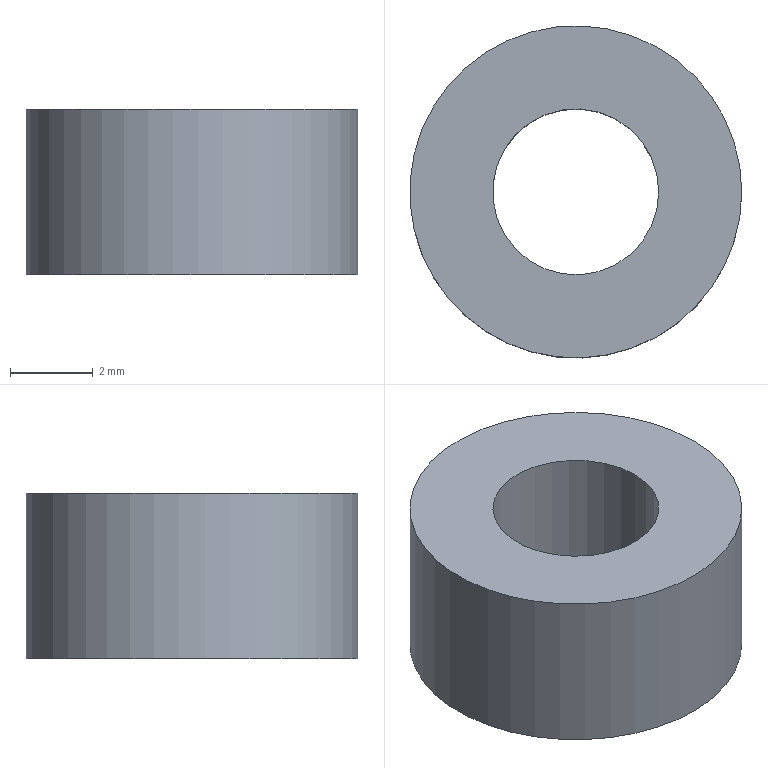Component | NX | LARGE_WASHER | 1 solid | 4 faces | box 8 x 8 x 4 mm | volume 151 mm3 | cylinder 2 | plane 2 | commonest cylinder face diameters 8 x1 4 x1
STEP:
#1=CARTESIAN_POINT('',(0.,0.,0.));
#2=DIRECTION('',(0.,0.,1.));
#3=DIRECTION('',(1.,0.,0.));
#4=AXIS2_PLACEMENT_3D('',#1,#2,#3);
#5=CARTESIAN_POINT('',(4.,23.,122.5));
#6=VERTEX_POINT('',#5);
#7=CARTESIAN_POINT('',(-0.,23.,122.5));
#8=DIRECTION('',(0.,0.,1.));
#9=DIRECTION('',(1.,0.,0.));
#10=AXIS2_PLACEMENT_3D('',#7,#8,#9);
#11=CIRCLE('',#10,4.);
#12=CARTESIAN_POINT('',(-0.,23.,122.5));
#13=DIRECTION('',(0.,0.,1.));
#14=DIRECTION('',(-1.,0.,0.));
#15=AXIS2_PLACEMENT_3D('',#12,#13,#14);
#16=CYLINDRICAL_SURFACE('',#15,4.);
#17=CARTESIAN_POINT('',(3.142,0.));
#18=DIRECTION('',(1.,0.));
#19=VECTOR('',#18,1.);
#20=LINE('',#17,#19);
#21=(GEOMETRIC_REPRESENTATION_CONTEXT(2)PARAMETRIC_REPRESENTATION_CONTEXT()REPRESENTATION_CONTEXT('',''));
#22=DEFINITIONAL_REPRESENTATION('',(#20),#21);
#23=PCURVE('',#16,#22);
#24=CARTESIAN_POINT('',(-0.,23.,122.5));
#25=DIRECTION('',(0.,0.,1.));
#26=DIRECTION('',(-1.,0.,0.));
#27=AXIS2_PLACEMENT_3D('',#24,#25,#26);
#28=PLANE('',#27);
#29=CARTESIAN_POINT('',(0.,0.));
#30=DIRECTION('',(-1.,0.));
#31=AXIS2_PLACEMENT_2D('',#29,#30);
#32=CIRCLE('',#31,4.);
#33=(GEOMETRIC_REPRESENTATION_CONTEXT(2)PARAMETRIC_REPRESENTATION_CONTEXT()REPRESENTATION_CONTEXT('',''));
#34=DEFINITIONAL_REPRESENTATION('',(#32),#33);
#35=PCURVE('',#28,#34);
#36=SURFACE_CURVE('',#11,(#23,#35),.PCURVE_S1.);
#37=EDGE_CURVE('',#6,#6,#36,.T.);
#38=ORIENTED_EDGE('',*,*,#37,.T.);
#39=CARTESIAN_POINT('',(4.,23.,126.5));
#40=VERTEX_POINT('',#39);
#41=CARTESIAN_POINT('',(4.,23.,122.5));
#42=CARTESIAN_POINT('',(4.,23.,126.5));
#43=B_SPLINE_CURVE_WITH_KNOTS('',1,(#41,#42),.UNSPECIFIED.,.F.,.F.,(2,2),(0.,4.),.PIECEWISE_BEZIER_KNOTS.);
#44=CARTESIAN_POINT('',(9.425,0.));
#45=DIRECTION('',(0.,1.));
#46=VECTOR('',#45,1.);
#47=LINE('',#44,#46);
#48=(GEOMETRIC_REPRESENTATION_CONTEXT(2)PARAMETRIC_REPRESENTATION_CONTEXT()REPRESENTATION_CONTEXT('',''));
#49=DEFINITIONAL_REPRESENTATION('',(#47),#48);
#50=PCURVE('',#16,#49);
#51=CARTESIAN_POINT('',(3.142,0.));
#52=DIRECTION('',(0.,1.));
#53=VECTOR('',#52,1.);
#54=LINE('',#51,#53);
#55=(GEOMETRIC_REPRESENTATION_CONTEXT(2)PARAMETRIC_REPRESENTATION_CONTEXT()REPRESENTATION_CONTEXT('',''));
#56=DEFINITIONAL_REPRESENTATION('',(#54),#55);
#57=PCURVE('',#16,#56);
#58=SEAM_CURVE('',#43,(#50,#57),.PCURVE_S1.);
#59=EDGE_CURVE('',#6,#40,#58,.T.);
#60=ORIENTED_EDGE('',*,*,#59,.T.);
#61=CARTESIAN_POINT('',(-0.,23.,126.5));
#62=DIRECTION('',(0.,0.,1.));
#63=DIRECTION('',(1.,0.,0.));
#64=AXIS2_PLACEMENT_3D('',#61,#62,#63);
#65=CIRCLE('',#64,4.);
#66=CARTESIAN_POINT('',(3.142,4.));
#67=DIRECTION('',(1.,0.));
#68=VECTOR('',#67,1.);
#69=LINE('',#66,#68);
#70=(GEOMETRIC_REPRESENTATION_CONTEXT(2)PARAMETRIC_REPRESENTATION_CONTEXT()REPRESENTATION_CONTEXT('',''));
#71=DEFINITIONAL_REPRESENTATION('',(#69),#70);
#72=PCURVE('',#16,#71);
#73=CARTESIAN_POINT('',(-0.,23.,126.5));
#74=DIRECTION('',(0.,0.,1.));
#75=DIRECTION('',(-1.,0.,0.));
#76=AXIS2_PLACEMENT_3D('',#73,#74,#75);
#77=PLANE('',#76);
#78=CARTESIAN_POINT('',(0.,0.));
#79=DIRECTION('',(-1.,0.));
#80=AXIS2_PLACEMENT_2D('',#78,#79);
#81=CIRCLE('',#80,4.);
#82=(GEOMETRIC_REPRESENTATION_CONTEXT(2)PARAMETRIC_REPRESENTATION_CONTEXT()REPRESENTATION_CONTEXT('',''));
#83=DEFINITIONAL_REPRESENTATION('',(#81),#82);
#84=PCURVE('',#77,#83);
#85=SURFACE_CURVE('',#65,(#72,#84),.PCURVE_S1.);
#86=EDGE_CURVE('',#40,#40,#85,.T.);
#87=ORIENTED_EDGE('',*,*,#86,.F.);
#88=ORIENTED_EDGE('',*,*,#59,.F.);
#89=EDGE_LOOP('',(#38,#60,#87,#88));
#90=FACE_BOUND('',#89,.T.);
#91=ADVANCED_FACE('',(#90),#16,.T.);
#92=CARTESIAN_POINT('',(2.,23.,122.5));
#93=VERTEX_POINT('',#92);
#94=CARTESIAN_POINT('',(-0.,23.,122.5));
#95=DIRECTION('',(0.,0.,1.));
#96=DIRECTION('',(1.,0.,0.));
#97=AXIS2_PLACEMENT_3D('',#94,#95,#96);
#98=CIRCLE('',#97,2.);
#99=CARTESIAN_POINT('',(-0.,23.,122.5));
#100=DIRECTION('',(0.,0.,1.));
#101=DIRECTION('',(-1.,0.,0.));
#102=AXIS2_PLACEMENT_3D('',#99,#100,#101);
#103=CYLINDRICAL_SURFACE('',#102,2.);
#104=CARTESIAN_POINT('',(3.142,0.));
#105=DIRECTION('',(1.,0.));
#106=VECTOR('',#105,1.);
#107=LINE('',#104,#106);
#108=(GEOMETRIC_REPRESENTATION_CONTEXT(2)PARAMETRIC_REPRESENTATION_CONTEXT()REPRESENTATION_CONTEXT('',''));
#109=DEFINITIONAL_REPRESENTATION('',(#107),#108);
#110=PCURVE('',#103,#109);
#111=CARTESIAN_POINT('',(0.,0.));
#112=DIRECTION('',(-1.,0.));
#113=AXIS2_PLACEMENT_2D('',#111,#112);
#114=CIRCLE('',#113,2.);
#115=(GEOMETRIC_REPRESENTATION_CONTEXT(2)PARAMETRIC_REPRESENTATION_CONTEXT()REPRESENTATION_CONTEXT('',''));
#116=DEFINITIONAL_REPRESENTATION('',(#114),#115);
#117=PCURVE('',#28,#116);
#118=SURFACE_CURVE('',#98,(#110,#117),.PCURVE_S1.);
#119=EDGE_CURVE('',#93,#93,#118,.T.);
#120=ORIENTED_EDGE('',*,*,#119,.T.);
#121=CARTESIAN_POINT('',(2.,23.,126.5));
#122=VERTEX_POINT('',#121);
#123=CARTESIAN_POINT('',(2.,23.,122.5));
#124=CARTESIAN_POINT('',(2.,23.,126.5));
#125=B_SPLINE_CURVE_WITH_KNOTS('',1,(#123,#124),.UNSPECIFIED.,.F.,.F.,(2,2),(0.,4.),.PIECEWISE_BEZIER_KNOTS.);
#126=CARTESIAN_POINT('',(9.425,0.));
#127=DIRECTION('',(0.,1.));
#128=VECTOR('',#127,1.);
#129=LINE('',#126,#128);
#130=(GEOMETRIC_REPRESENTATION_CONTEXT(2)PARAMETRIC_REPRESENTATION_CONTEXT()REPRESENTATION_CONTEXT('',''));
#131=DEFINITIONAL_REPRESENTATION('',(#129),#130);
#132=PCURVE('',#103,#131);
#133=CARTESIAN_POINT('',(3.142,0.));
#134=DIRECTION('',(0.,1.));
#135=VECTOR('',#134,1.);
#136=LINE('',#133,#135);
#137=(GEOMETRIC_REPRESENTATION_CONTEXT(2)PARAMETRIC_REPRESENTATION_CONTEXT()REPRESENTATION_CONTEXT('',''));
#138=DEFINITIONAL_REPRESENTATION('',(#136),#137);
#139=PCURVE('',#103,#138);
#140=SEAM_CURVE('',#125,(#132,#139),.PCURVE_S1.);
#141=EDGE_CURVE('',#93,#122,#140,.T.);
#142=ORIENTED_EDGE('',*,*,#141,.T.);
#143=CARTESIAN_POINT('',(-0.,23.,126.5));
#144=DIRECTION('',(0.,0.,1.));
#145=DIRECTION('',(1.,0.,0.));
#146=AXIS2_PLACEMENT_3D('',#143,#144,#145);
#147=CIRCLE('',#146,2.);
#148=CARTESIAN_POINT('',(3.142,4.));
#149=DIRECTION('',(1.,0.));
#150=VECTOR('',#149,1.);
#151=LINE('',#148,#150);
#152=(GEOMETRIC_REPRESENTATION_CONTEXT(2)PARAMETRIC_REPRESENTATION_CONTEXT()REPRESENTATION_CONTEXT('',''));
#153=DEFINITIONAL_REPRESENTATION('',(#151),#152);
#154=PCURVE('',#103,#153);
#155=CARTESIAN_POINT('',(0.,0.));
#156=DIRECTION('',(-1.,0.));
#157=AXIS2_PLACEMENT_2D('',#155,#156);
#158=CIRCLE('',#157,2.);
#159=(GEOMETRIC_REPRESENTATION_CONTEXT(2)PARAMETRIC_REPRESENTATION_CONTEXT()REPRESENTATION_CONTEXT('',''));
#160=DEFINITIONAL_REPRESENTATION('',(#158),#159);
#161=PCURVE('',#77,#160);
#162=SURFACE_CURVE('',#147,(#154,#161),.PCURVE_S1.);
#163=EDGE_CURVE('',#122,#122,#162,.T.);
#164=ORIENTED_EDGE('',*,*,#163,.F.);
#165=ORIENTED_EDGE('',*,*,#141,.F.);
#166=EDGE_LOOP('',(#120,#142,#164,#165));
#167=FACE_BOUND('',#166,.F.);
#168=ADVANCED_FACE('',(#167),#103,.F.);
#169=ORIENTED_EDGE('',*,*,#37,.F.);
#170=EDGE_LOOP('',(#169));
#171=FACE_BOUND('',#170,.T.);
#172=ORIENTED_EDGE('',*,*,#119,.T.);
#173=EDGE_LOOP('',(#172));
#174=FACE_BOUND('',#173,.T.);
#175=ADVANCED_FACE('',(#171,#174),#28,.F.);
#176=ORIENTED_EDGE('',*,*,#86,.T.);
#177=EDGE_LOOP('',(#176));
#178=FACE_BOUND('',#177,.T.);
#179=ORIENTED_EDGE('',*,*,#163,.F.);
#180=EDGE_LOOP('',(#179));
#181=FACE_BOUND('',#180,.T.);
#182=ADVANCED_FACE('',(#178,#181),#77,.T.);
#183=CLOSED_SHELL('',(#91,#168,#175,#182));
#184=MANIFOLD_SOLID_BREP('',#183);
#185=(LENGTH_UNIT()NAMED_UNIT(*)SI_UNIT(.MILLI.,.METRE.));
#186=UNCERTAINTY_MEASURE_WITH_UNIT(LENGTH_MEASURE(0.00001),#185,'','');
#187=(NAMED_UNIT(*)PLANE_ANGLE_UNIT()SI_UNIT($,.RADIAN.));
#188=(NAMED_UNIT(*)SI_UNIT($,.STERADIAN.)SOLID_ANGLE_UNIT());
#189=(GEOMETRIC_REPRESENTATION_CONTEXT(3)GLOBAL_UNCERTAINTY_ASSIGNED_CONTEXT((#186))GLOBAL_UNIT_ASSIGNED_CONTEXT((#185,#187,#188))REPRESENTATION_CONTEXT('',''));
#190=ADVANCED_BREP_SHAPE_REPRESENTATION('',(#4,#184),#189);